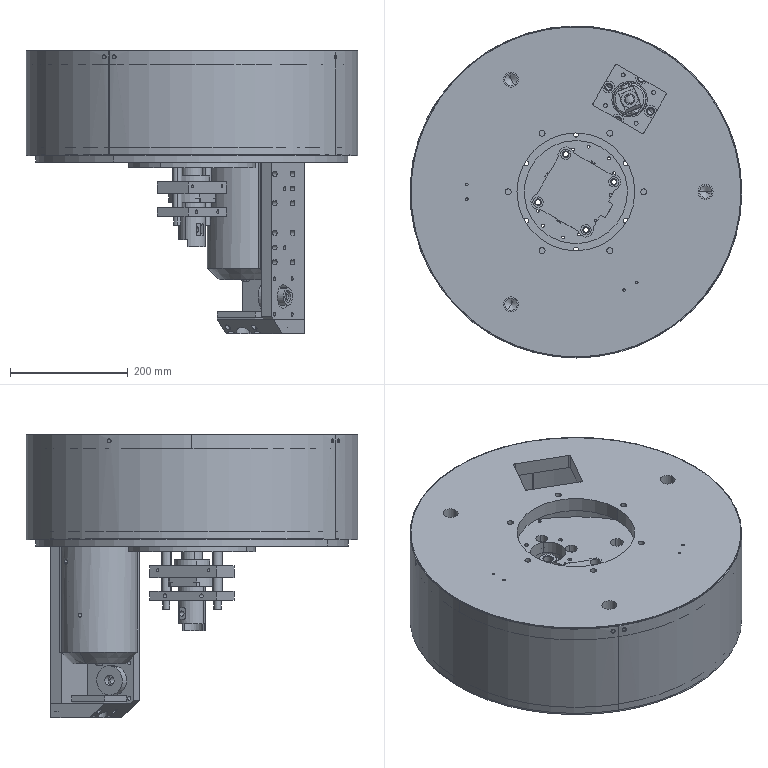Assembly | SolidWorks | mm | 29 component files | 31 solids | 1237 faces | box 563 x 563 x 481.5 mm | volume 16999880 mm3 | cylinder 695 | plane 385 | cone 123 | torus 28 | spline 6 | commonest cylinder face diameters 6.8 x78 5 x62 9 x50 7 x36 11 x36 6 x35 8.5 x32 8.8 x24
Bill of materials:
KLHFH001LocatingPlate | 1 | AISI Type A2 Tool Steel | Square flat plate of moderate thickness with one large central through hole and six smaller through holes in two parallel rows of three, one row on each side of the central hole.
KLHFH002Turntable | 1 | Plain Carbon Steel | Thin circular disc with a large central through hole, a smaller offset hole ringed by a pattern of smaller holes, three counterbored holes near the rim, several other medium holes, and small holes scattered near the edge. The side profile shows a step at the perimeter: the top layer is slightly larger in diameter than the bottom layer.
KLHFH002Turntable-1 | 1 | Plain Carbon Steel | Flat circular disc of uniform thickness with a large central through hole, a square cutout with rounded corners offset from center, eight small holes evenly spaced around the central bore, three larger holes near the rim, and two pairs of very small holes.
KLHFH003PinSlider-SymmetricPart(2) | 1 | Plain Carbon Steel | Tall prismatic block whose cross-section is a partial circle cut by two flat faces meeting at an angle. It has a central axial bore, four holes on the end face around the bore, rows of small holes on the flat side faces, and chamfered or rounded transitions at the lower end.
KLHFH004LocatingSeatConnectingFixingPlate-SymmetricPart | 1 | Plain Carbon Steel | L-shaped angle bracket with two flat legs at roughly 90 degrees and unequal leg widths. Both legs carry many holes, including slotted (elongated) holes and small round holes. One leg has a larger round hole near one end that appears to be crossed by a small side hole, and one corner is chamfered.
KLHFH005_18LocatingPin-Copy | 1 | AISI Type A2 Tool Steel | Turned stepped pin with a circular flange head pierced by four through holes, a non-circular section with flats or notches below the flange, a cylindrical shank, a circumferential groove near the lower end, and a short cylindrical section ending in a conical tip.
KLHFH006_18LocatingPinFixingSeat | 1 | Plain Carbon Steel | Stepped cylindrical body, larger diameter on top and smaller below, with small edge chamfers. A flat rectangular tab with a rounded end and a round through hole projects from the top face, forming an eye or lug.
KLHFH007_18LocatingPinSeatBrassSleeve | 1 | Brass | Thin-walled cylindrical tube or sleeve, open at both ends, with a shallow circumferential groove on the outside near mid-length.
KLHFH008LimitPlate-SymmetricPart | 1 | Plain Carbon Steel | Thick square plate with one edge beveled at an angle. It has one large through hole and roughly a dozen smaller through holes of two or more sizes spread across the face.
KLHFH014_60HighGuideRod | 3 | Plain Carbon Steel | Plain cylindrical spacer or bushing with one central axial hole.
KLHFH017AdjustmentShim | 2 | Plain Carbon Steel | Thin flat rectangular strip with six open-ended U-shaped slots along one long edge, in two groups of three separated by a solid section.
KLHFH018AdjustmentShim | 1 | AISI 304 | Thin flat roughly square plate with three parallel open-ended slots from one edge: a wide slot in the middle with a rounded end, and a narrower slot with a rounded end on each side.
KLHFH019EjectorPlate | 1 | 6061 Alloy | Hollow flanged bushing: a short large-diameter cylindrical flange with a smaller coaxial cylindrical boss, through bore, and a counterbore at the boss end.
KLHFH026SynchronousBeltCover | 1 | AISI 304 | Thin-walled open cylindrical band (ring/sleeve) with a few small radial holes near one edge, spaced unevenly around the circumference.
PressureReducingValveHolder | 1 |  | Bent sheet bracket in an L shape with a bend radius: a flat rectangular flange with two small holes, and a perpendicular leg with a rounded end, one large round hole and a rectangular window near the bend.
A_CDQ2B100-15DM(0) | 1 |  | Compact square-section prismatic body with chamfered/notched corners holding four axial through holes, longitudinal grooves along the sides, two side ports, and a cylindrical rod with a shoulder sticking out from one end face.
KLHFH002Turntable-2 | 1 | Plain Carbon Steel | Flat circular plate with a raised concentric annular step on one face, a large central through hole, and many smaller through holes of several sizes in an irregular pattern, with larger holes near the outer rim.
KLHFH009_38LocatingPin | 1 | AISI Type A2 Tool Steel | Flanged cylindrical body: a D-shaped/truncated-oval flange with four holes, a raised circular boss on the flange face, a cylindrical shank with flat spot-faced pads and cross holes, and a stepped or partly cut-away end.
KLHFH010_38LocatingPinFixingSeat | 1 | Plain Carbon Steel | Rectangular block plate with two large counterbores and through holes near the ends, a central hole, several smaller holes on the top face, and holes in the long side faces.
KLHFH011100CylinderConnectingSeatSLDPRT | 1 | Plain Carbon Steel | Flanged hub: a circular flange disc with four evenly spaced through holes and a coaxial cylindrical boss, with a large through bore.
KLHFH012_16GuideRodSLDPRT | 2 | Plain Carbon Steel | Slender stepped cylindrical pin/tube: a longer large-diameter section and a shorter reduced-diameter section, with an axial hole at the larger end.
KLHFH015_38LocatingPinLimitPlate | 1 | Plain Carbon Steel | Rectangular plate with a large central through hole, two pairs of smaller holes (one larger and one smaller hole in each pair) toward the ends, and holes in the long side faces.
KLHFH016_16CopperSleeve | 2 | Brass | Thick-walled cylindrical ring/spacer with a large central bore and a semicircular groove around the middle of its outer surface.
Y-G05 | 1 | Plain Carbon Steel | Clevis-type fork body with two parallel rounded lugs joined by a cross pin, a squared upper block with chamfered edges, and a cylindrical boss with a bore on top.
Mates:
1. coincident | KLHFH002Turntable-1-1 plane at (0, 0, 0) dir (0, 1, 0) | assembly plane at (0, 0, 0) dir (0, 1, 0)
2. coincident | KLHFH002Turntable-1-1 plane at (0, 0, 0) dir (1, 0, 0) | assembly plane at (0, 0, 0) dir (1, 0, 0)
3. coincident | KLHFH002Turntable-1-1 plane at (0, 0, 0) dir (0, 0, 1) | assembly plane at (0, 0, 0) dir (0, 0, 1)
4. concentric | KLHFH002Turntable-1-1 face at (220, 0, 12.5) dir (0, 0, 1) r 12.75 | KLHFH014_60HighGuideRod-1 face at (220, 0, -7.5) dir (0, 0, -1) r 30
5. coincident | KLHFH002Turntable-1-1 face at (220, 0, -7.5) dir (0, 0, -1) | KLHFH014_60HighGuideRod-1 face at (220, 0, -7.5) dir (0, 0, 1)
6. coincident | KLHFH002Turntable-1-1 face at (0, 0, -12.5) dir (0, 0, -1) | PressureReducingValveHolder-1 face at (-168, -50, -12.5) dir (0, 0, 1)
7. concentric | KLHFH002Turntable-1-1 face at (0, 0, -12.5) dir (0, 0, 1) r 100 | KLHFH002Turntable-1 face at (0, 0, -152.5) dir (0, 0, -1) r 87.5
8. concentric | KLHFH014_60HighGuideRod-1 face at (220, 0, -7.5) dir (0, 0, -1) r 30 | KLHFH002Turntable-1 face at (220, 0, -157.5) dir (0, 0, 1) r 30
9. coincident | KLHFH014_60HighGuideRod-1 face at (220, 0, -157.5) dir (0, 0, -1) | KLHFH002Turntable-1 face at (220, 0, -157.5) dir (0, 0, 1)
10. coincident | KLHFH002Turntable-1 face at (0, 0, -177.5) dir (0, 0, -1) | KLHFH017AdjustmentShim-2 face at (116.133, 95.148, -177.5) dir (0, 0, 1)
11. coincident | KLHFH005_18LocatingPin-Copy-1 face at (91, 157.617, -335.5) dir (0, 0, 1) | KLHFH006_18LocatingPinFixingSeat-1 face at (91, 157.617, -335.5) dir (0, 0, -1)
12. concentric | KLHFH005_18LocatingPin-Copy-1 face at (91, 157.617, -345.5) dir (0, 0, -1) r 9 | KLHFH006_18LocatingPinFixingSeat-1 face at (91, 157.617, -320.5) dir (0, 0, -1) r 6
13. concentric | KLHFH005_18LocatingPin-Copy-1 face at (85.856, 170.637, -345.5) dir (0, 0, -1) r 3 | KLHFH006_18LocatingPinFixingSeat-1 face at (85.856, 170.637, -335.5) dir (0, 0, -1) r 1.65
14. concentric | KLHFH006_18LocatingPinFixingSeat-1 face at (101.104, 132.04, -206) dir (-0.3674, 0.9301, 0) r 7 | Y-G05-1 face at (95.041, 147.386, -206) dir (0.3674, -0.9301, 0) r 7
15. concentric | KLHFH006_18LocatingPinFixingSeat-1 face at (91, 157.617, -226) dir (0, 0, -1) r 27.5 | Y-G05-1 face at (91, 157.617, -186) dir (0, 0, 1) r 7.645
16. coincident | KLHFH018AdjustmentShim-1 face at (90.792, 157.737, -441) dir (0, 0, 1) | KLHFH001LocatingPlate-1 face at (91, 157.617, -441) dir (0, 0, -1)
17. coincident | KLHFH018AdjustmentShim-1 face at (42.749, 148.524, -441) dir (-0.5, -0.866, 0) | KLHFH001LocatingPlate-1 face at (107.043, 111.404, -431) dir (-0.5, -0.866, 0)
18. concentric | KLHFH002Turntable-1 face at (0, 0, -152.5) dir (0, 0, -1) r 87.5 | SpindleFixtureAssemblyLeft-1/KLHFH002Turntable-2-1 face at (0, 0, -177.5) dir (0, 0, 1) r 87.5
19. coincident | KLHFH002Turntable-1 face at (0, 0, -177.5) dir (0, 0, -1) | SpindleFixtureAssemblyLeft-1/KLHFH002Turntable-2-1 face at (0, 0, -177.5) dir (0, 0, 1)
20. concentric | KLHFH002Turntable-1 face at (84.437, 48.75, -177.5) dir (0, 0, -1) r 4.25 | SpindleFixtureAssemblyLeft-1/KLHFH002Turntable-2-1 face at (84.437, 48.75, -187.5) dir (0, 0, -1) r 5.5
21. concentric | KLHFH002Turntable-1 face at (91, 157.617, -152.5) dir (0, 0, -1) r 30 | KLHFH003PinSlider-SymmetricPart(2)-1 face at (91, 157.617, -344.5) dir (0, 0, 1) r 32.5
22. coincident | KLHFH002Turntable-1 face at (91, 157.617, -174.5) dir (0, 0, -1) | KLHFH003PinSlider-SymmetricPart(2)-1 face at (91, 157.617, -174.5) dir (0, 0, 1)
23. concentric | KLHFH002Turntable-1 face at (111.5, 193.124, -152.5) dir (0, 0, 1) r 10 | KLHFH003PinSlider-SymmetricPart(2)-1 face at (111.5, 193.124, -174.5) dir (0, 0, 1) r 5.1
24. coincident | KLHFH017AdjustmentShim-1 face at (80.031, 221.684, -357.5) dir (-0.5, -0.866, 0) | KLHFH003PinSlider-SymmetricPart(2)-1 face at (151.969, 180.151, -174.5) dir (0.5, 0.866, 0)
25. coincident | KLHFH017AdjustmentShim-1 face at (81.531, 224.283, -357.5) dir (-0.866, 0.5, 0) | KLHFH003PinSlider-SymmetricPart(2)-1 edge at (80.031, 221.684, -174.5) dir (0, 0, -1)
26. coincident | KLHFH002Turntable-1 face at (0, 0, -177.5) dir (0, 0, -1) | KLHFH017AdjustmentShim-1 face at (81.531, 224.283, -177.5) dir (0, 0, 1)
27. coincident | KLHFH017AdjustmentShim-2 face at (113.535, 96.648, -177.5) dir (-0.866, 0.5, 0) | KLHFH003PinSlider-SymmetricPart(2)-1 face at (113.535, 96.648, -174.5) dir (0.866, -0.5, 0)
28. coincident | KLHFH017AdjustmentShim-2 face at (116.133, 95.148, -177.5) dir (-0.5, -0.866, 0) | KLHFH003PinSlider-SymmetricPart(2)-1 edge at (113.535, 96.648, -174.5) dir (0, 0, -1)
29. coincident | KLHFH017AdjustmentShim-1 face at (81.531, 224.283, -357.5) dir (0.5, 0.866, 0) | KLHFH004LocatingSeatConnectingFixingPlate-SymmetricPart-1 face at (163.399, 177.016, -444) dir (-0.5, -0.866, 0)
30. coincident | KLHFH017AdjustmentShim-2 face at (116.133, 95.148, -177.5) dir (0.866, -0.5, 0) | KLHFH004LocatingSeatConnectingFixingPlate-SymmetricPart-1 face at (163.399, 177.016, -444) dir (-0.866, 0.5, 0)
31. tangent | KLHFH003PinSlider-SymmetricPart(2)-1 face at (92.617, 214.418, -212.5) dir (0.5, 0.866, 0) r 4 | KLHFH004LocatingSeatConnectingFixingPlate-SymmetricPart-1 face at (107.148, 232.586, -216.5) dir (0, 0, 1)
32. concentric | KLHFH004LocatingSeatConnectingFixingPlate-SymmetricPart-1 face at (177.054, 180.667, -444) dir (0, 0, -1) r 4 | KLHFH008LimitPlate-SymmetricPart-1 face at (177.054, 180.667, -444) dir (0, 0, 1) r 4
33. coincident | KLHFH004LocatingSeatConnectingFixingPlate-SymmetricPart-1 face at (163.399, 177.016, -444) dir (0, 0, -1) | KLHFH008LimitPlate-SymmetricPart-1 face at (115.588, 164.205, -444) dir (0, 0, 1)
34. concentric | KLHFH004LocatingSeatConnectingFixingPlate-SymmetricPart-1 face at (129.426, 208.173, -444) dir (0, 0, -1) r 4 | KLHFH008LimitPlate-SymmetricPart-1 face at (129.426, 208.173, -444) dir (0, 0, 1) r 4
35. coincident | KLHFH018AdjustmentShim-1 face at (90.792, 157.737, -444) dir (0, 0, -1) | KLHFH008LimitPlate-SymmetricPart-1 face at (115.588, 164.205, -444) dir (0, 0, 1)
36. concentric | KLHFH001LocatingPlate-1 face at (76, 183.597, -441) dir (0, 0, -1) r 3 | KLHFH008LimitPlate-SymmetricPart-1 face at (76, 183.597, -444) dir (0, 0, 1) r 4.5
37. concentric | KLHFH001LocatingPlate-1 face at (61, 157.617, -441) dir (0, 0, -1) r 3 | KLHFH008LimitPlate-SymmetricPart-1 face at (61, 157.617, -444) dir (0, 0, 1) r 4.5
38. concentric | KLHFH007_18LocatingPinSeatBrassSleeve-1 face at (91, 157.617, -244.5) dir (0, 0, -1) r 32.5 | KLHFH006_18LocatingPinFixingSeat-1 face at (91, 157.617, -271) dir (0, 0, -1) r 22.5
39. coincident | KLHFH007_18LocatingPinSeatBrassSleeve-1 face at (91, 157.617, -344.5) dir (0, 0, -1) | KLHFH003PinSlider-SymmetricPart(2)-1 edge at (91, 157.617, -344.5) dir (0, 0, 1) r 32.5
40. concentric | KLHFH002Turntable-1-1 face at (-185, -12.45, -12.5) dir (0, 0, -1) r 2.1 | PressureReducingValveHolder-1 face at (-185, -12.45, -15.5) dir (0, 0, -1) r 3.5
41. concentric | KLHFH002Turntable-1-1 face at (0, 0, 12.5) dir (0, 0, -1) r 280 | KLHFH026SynchronousBeltCover-1 face at (0, 0, -166.5) dir (0, 0, 1) r 281.5
42. concentric | KLHFH002Turntable-1 face at (144.668, 231.517, -165) dir (0, 0, -1) r 2.5 | KLHFH026SynchronousBeltCover-1 face at (144.668, 231.517, -166.5) dir (0, 0, -1) r 3.5
43. coincident | KLHFH002Turntable-1 face at (0, 0, -165) dir (0, 0, -1) | KLHFH026SynchronousBeltCover-1 face at (0, 0, -165) dir (0, 0, 1)
44. coincident | KLHFH019EjectorPlate-1 face at (137.649, 132.416, -405.5) dir (0.866, -0.5, 0) | KLHFH004LocatingSeatConnectingFixingPlate-SymmetricPart-1 face at (163.399, 177.016, -444) dir (-0.866, 0.5, 0)
45. concentric | KLHFH002Turntable-2-1 face at (-27.615, -2.762, 205) dir (0, 0, 1) r 35 | A_CDQ2B100-15DM(0)-1 face at (-27.615, -2.762, 247.835) dir (0, 0, 1) r 13
46. concentric | KLHFH002Turntable-2-1 face at (19.385, -49.762, 205) dir (0, 0, -1) r 4.25 | A_CDQ2B100-15DM(0)-1 face at (19.385, -49.762, 191.5) dir (0, 0, 1) r 8.75
47. coincident | KLHFH002Turntable-2-1 face at (-27.615, -2.762, 205) dir (0, 0, -1) | A_CDQ2B100-15DM(0)-1 face at (-86.115, -61.262, 205) dir (0, 0, 1)
48. concentric | KLHFH002Turntable-2-1 face at (-77.615, -2.762, 222) dir (0, 0, 1) r 8 | KLHFH012_16GuideRodSLDPRT-1 face at (-77.615, -2.762, 292) dir (0, 0, -1) r 8
49. coincident | KLHFH002Turntable-2-1 face at (-77.615, -2.762, 222) dir (0, 0, 1) | KLHFH012_16GuideRodSLDPRT-1 face at (-77.615, -2.762, 222) dir (0, 0, -1)
50. concentric | KLHFH002Turntable-2-1 face at (22.385, -2.762, 222) dir (0, 0, 1) r 8 | KLHFH012_16GuideRodSLDPRT-2 face at (22.385, -2.762, 292) dir (0, 0, -1) r 8
51. coincident | KLHFH002Turntable-2-1 face at (22.385, -2.762, 222) dir (0, 0, 1) | KLHFH012_16GuideRodSLDPRT-2 face at (22.385, -2.762, 222) dir (0, 0, -1)
52. coincident | A_CDQ2B100-15DM(0)-1 face at (-15.132, -15.097, 248.5) dir (0, 0, 1) | KLHFH011100CylinderConnectingSeatSLDPRT-1 face at (-27.615, -2.762, 248.5) dir (0, 0, 1)
53. concentric | A_CDQ2B100-15DM(0)-1 face at (-27.615, -2.762, 247.835) dir (0, 0, 1) r 13 | KLHFH011100CylinderConnectingSeatSLDPRT-1 face at (-27.615, -2.762, 223.5) dir (0, 0, -1) r 13
54. concentric | KLHFH010_38LocatingPinFixingSeat-1 face at (22.385, -2.762, 263.5) dir (0, 0, -1) r 12.5 | KLHFH016_16CopperSleeve-1 face at (22.385, -2.762, 263.5) dir (0, 0, -1) r 12.5
55. coincident | KLHFH010_38LocatingPinFixingSeat-1 face at (22.385, -2.762, 263.5) dir (0, 0, -1) | KLHFH016_16CopperSleeve-1 face at (22.385, -2.762, 263.5) dir (0, 0, 1)
56. concentric | KLHFH010_38LocatingPinFixingSeat-1 face at (-77.615, -2.762, 263.5) dir (0, 0, -1) r 12.5 | KLHFH016_16CopperSleeve-2 face at (-77.615, -2.762, 263.5) dir (0, 0, -1) r 12.5
57. coincident | KLHFH010_38LocatingPinFixingSeat-1 face at (-77.615, -2.762, 263.5) dir (0, 0, -1) | KLHFH016_16CopperSleeve-2 face at (-77.615, -2.762, 263.5) dir (0, 0, 1)
58. concentric | KLHFH012_16GuideRodSLDPRT-1 face at (-77.615, -2.762, 292) dir (0, 0, -1) r 8 | KLHFH016_16CopperSleeve-2 face at (-77.615, -2.762, 263.5) dir (0, 0, -1) r 8
59. concentric | KLHFH012_16GuideRodSLDPRT-2 face at (22.385, -2.762, 292) dir (0, 0, -1) r 8 | KLHFH016_16CopperSleeve-1 face at (22.385, -2.762, 263.5) dir (0, 0, -1) r 8
60. concentric | KLHFH011100CylinderConnectingSeatSLDPRT-1 face at (-44.409, -19.555, 238.5) dir (0, 0, -1) r 3.5 | KLHFH010_38LocatingPinFixingSeat-1 face at (-44.409, -19.555, 248.5) dir (0, 0, -1) r 2.5
61. coincident | KLHFH011100CylinderConnectingSeatSLDPRT-1 face at (-27.615, -2.762, 248.5) dir (0, 0, 1) | KLHFH010_38LocatingPinFixingSeat-1 face at (-27.615, -2.762, 248.5) dir (0, 0, -1)
62. concentric | KLHFH010_38LocatingPinFixingSeat-1 face at (-27.615, -2.762, 263.5) dir (0, 0, 1) r 22.5 | KLHFH015_38LocatingPinLimitPlate-1 face at (-27.615, -2.762, 292) dir (0, 0, 1) r 23.5
63. concentric | KLHFH012_16GuideRodSLDPRT-2 face at (22.385, -2.762, 292) dir (0, 0, -1) r 8 | KLHFH015_38LocatingPinLimitPlate-1 face at (22.385, -2.762, 307) dir (0, 0, -1) r 6.25
64. coincident | KLHFH012_16GuideRodSLDPRT-2 face at (22.385, -2.762, 292) dir (0, 0, 1) | KLHFH015_38LocatingPinLimitPlate-1 face at (-27.615, -2.762, 292) dir (0, 0, -1)
65. concentric | KLHFH010_38LocatingPinFixingSeat-1 face at (-27.615, -2.762, 263.5) dir (0, 0, 1) r 22.5 | KLHFH009_38LocatingPin-1 face at (-27.615, -2.762, 358.5) dir (0, 0, -1) r 22.5
66. concentric | KLHFH010_38LocatingPinFixingSeat-1 face at (-51.657, -26.803, 268.5) dir (0, 0, 1) r 2.5 | KLHFH009_38LocatingPin-1 face at (-51.657, -26.803, 283.5) dir (0, 0, 1) r 5.5
67. coincident | KLHFH010_38LocatingPinFixingSeat-1 face at (-27.615, -2.762, 268.5) dir (0, 0, 1) | KLHFH009_38LocatingPin-1 face at (-27.615, -2.762, 268.5) dir (0, 0, -1)